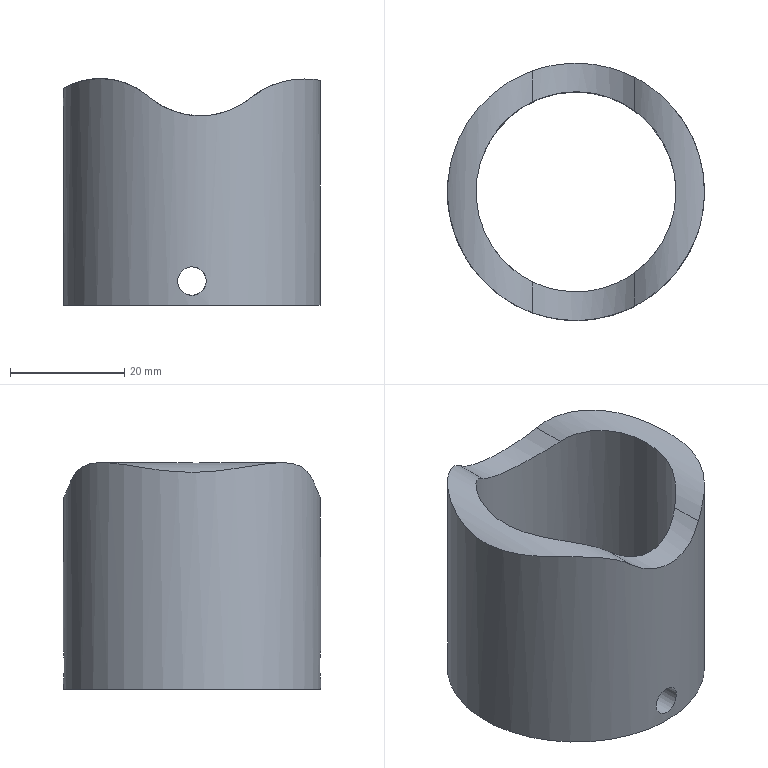Component | NX | PISTON | 1 solid | 9 faces | box 45 x 45 x 39.71 mm | volume 23430 mm3 | cylinder 8 | plane 1 | commonest cylinder face diameters 27.799 x2 5 x2 45 x1 35 x1 26.024 x1 29.489 x1
STEP:
#1=VALUE_REPRESENTATION_ITEM('',COUNT_MEASURE(0.));
#2=(LENGTH_UNIT()NAMED_UNIT(*)SI_UNIT(.MILLI.,.METRE.));
#3=UNCERTAINTY_MEASURE_WITH_UNIT(LENGTH_MEASURE(0.0508),#2,'','');
#4=(NAMED_UNIT(*)PLANE_ANGLE_UNIT()SI_UNIT($,.RADIAN.));
#5=PLANE_ANGLE_MEASURE_WITH_UNIT(PLANE_ANGLE_MEASURE(0.01745),#4);
#6=DIMENSIONAL_EXPONENTS(0.,0.,0.,0.,0.,0.,0.);
#7=(CONVERSION_BASED_UNIT('',#5)NAMED_UNIT(#6)PLANE_ANGLE_UNIT());
#8=(NAMED_UNIT(*)SI_UNIT($,.STERADIAN.)SOLID_ANGLE_UNIT());
#9=(GEOMETRIC_REPRESENTATION_CONTEXT(3)GLOBAL_UNCERTAINTY_ASSIGNED_CONTEXT((#3))GLOBAL_UNIT_ASSIGNED_CONTEXT((#2,#7,#8))REPRESENTATION_CONTEXT('',''));
#10=REPRESENTATION('',(#1),#9);
#11=VALUE_REPRESENTATION_ITEM('',COUNT_MEASURE(0.));
#12=REPRESENTATION('',(#11),#9);
#13=CARTESIAN_POINT('',(0.,0.,0.));
#14=DIRECTION('',(0.,0.,1.));
#15=DIRECTION('',(1.,0.,0.));
#16=AXIS2_PLACEMENT_3D('',#13,#14,#15);
#17=SHAPE_REPRESENTATION('',(#16),#9);
#18=CARTESIAN_POINT('',(2.606,67.362,109.935));
#19=VERTEX_POINT('',#18);
#20=CARTESIAN_POINT('',(2.606,67.362,109.935));
#21=CARTESIAN_POINT('',(2.606,67.362,110.214));
#22=CARTESIAN_POINT('',(2.558,67.368,110.497));
#23=CARTESIAN_POINT('',(2.466,67.377,110.76));
#24=CARTESIAN_POINT('',(2.374,67.387,111.023));
#25=CARTESIAN_POINT('',(2.235,67.401,111.273));
#26=CARTESIAN_POINT('',(2.062,67.416,111.491));
#27=CARTESIAN_POINT('',(1.888,67.431,111.71));
#28=CARTESIAN_POINT('',(1.674,67.447,111.902));
#29=CARTESIAN_POINT('',(1.437,67.461,112.051));
#30=CARTESIAN_POINT('',(1.2,67.475,112.2));
#31=CARTESIAN_POINT('',(0.9339,67.487,112.31));
#32=CARTESIAN_POINT('',(0.6604,67.494,112.373));
#33=CARTESIAN_POINT('',(0.388,67.5,112.435));
#34=CARTESIAN_POINT('',(0.1011,67.502,112.451));
#35=CARTESIAN_POINT('',(-0.1765,67.498,112.419));
#36=CARTESIAN_POINT('',(-0.4529,67.494,112.388));
#37=CARTESIAN_POINT('',(-0.7277,67.485,112.308));
#38=CARTESIAN_POINT('',(-0.9781,67.473,112.188));
#39=CARTESIAN_POINT('',(-1.229,67.461,112.067));
#40=CARTESIAN_POINT('',(-1.463,67.445,111.902));
#41=CARTESIAN_POINT('',(-1.66,67.43,111.705));
#42=CARTESIAN_POINT('',(-1.858,67.414,111.507));
#43=CARTESIAN_POINT('',(-2.025,67.398,111.273));
#44=CARTESIAN_POINT('',(-2.146,67.386,111.021));
#45=CARTESIAN_POINT('',(-2.268,67.373,110.768));
#46=CARTESIAN_POINT('',(-2.348,67.364,110.491));
#47=CARTESIAN_POINT('',(-2.379,67.361,110.213));
#48=CARTESIAN_POINT('',(-2.41,67.357,109.935));
#49=CARTESIAN_POINT('',(-2.394,67.359,109.649));
#50=CARTESIAN_POINT('',(-2.331,67.366,109.377));
#51=CARTESIAN_POINT('',(-2.269,67.373,109.106));
#52=CARTESIAN_POINT('',(-2.16,67.385,108.842));
#53=CARTESIAN_POINT('',(-2.012,67.399,108.607));
#54=CARTESIAN_POINT('',(-1.864,67.413,108.371));
#55=CARTESIAN_POINT('',(-1.673,67.43,108.157));
#56=CARTESIAN_POINT('',(-1.456,67.445,107.982));
#57=CARTESIAN_POINT('',(-1.237,67.46,107.807));
#58=CARTESIAN_POINT('',(-0.9845,67.474,107.668));
#59=CARTESIAN_POINT('',(-0.7198,67.484,107.575));
#60=CARTESIAN_POINT('',(-0.4557,67.494,107.483));
#61=CARTESIAN_POINT('',(-0.1718,67.5,107.435));
#62=CARTESIAN_POINT('',(0.1082,67.5,107.435));
#63=CARTESIAN_POINT('',(0.3867,67.5,107.435));
#64=CARTESIAN_POINT('',(0.6689,67.495,107.483));
#65=CARTESIAN_POINT('',(0.9316,67.485,107.575));
#66=CARTESIAN_POINT('',(1.194,67.476,107.667));
#67=CARTESIAN_POINT('',(1.444,67.462,107.806));
#68=CARTESIAN_POINT('',(1.662,67.447,107.979));
#69=CARTESIAN_POINT('',(1.881,67.432,108.153));
#70=CARTESIAN_POINT('',(2.072,67.416,108.367));
#71=CARTESIAN_POINT('',(2.221,67.402,108.603));
#72=CARTESIAN_POINT('',(2.371,67.388,108.84));
#73=CARTESIAN_POINT('',(2.481,67.376,109.107));
#74=CARTESIAN_POINT('',(2.543,67.369,109.38));
#75=CARTESIAN_POINT('',(2.585,67.365,109.562));
#76=CARTESIAN_POINT('',(2.606,67.362,109.749));
#77=CARTESIAN_POINT('',(2.606,67.362,109.935));
#78=B_SPLINE_CURVE_WITH_KNOTS('',3,(#20,#21,#22,#23,#24,#25,#26,#27,#28,#29,#30,#31,#32,#33,#34,#35,#36,#37,#38,#39,#40,#41,#42,#43,#44,#45,#46,#47,#48,#49,#50,#51,#52,#53,#54,#55,#56,#57,#58,#59,#60,#61,#62,#63,#64,#65,#66,#67,#68,#69,#70,#71,#72,#73,#74,#75,#76,#77),.UNSPECIFIED.,.T.,.F.,(1,3,3,3,3,3,3,3,3,3,3,3,3,3,3,3,3,3,3,3,3,1),(-0.0354,0.,0.05348,0.1069,0.1606,0.2144,0.268,0.3214,0.3749,0.4286,0.4824,0.5359,0.5892,0.6428,0.6966,0.7503,0.8037,0.8571,0.9108,0.9646,1.,1.053),.UNSPECIFIED.);
#79=EDGE_CURVE('',#19,#19,#78,.T.);
#80=ORIENTED_EDGE('',*,*,#79,.T.);
#81=EDGE_LOOP('',(#80));
#82=FACE_BOUND('',#81,.T.);
#83=CARTESIAN_POINT('',(0.1196,22.5,107.435));
#84=VERTEX_POINT('',#83);
#85=CARTESIAN_POINT('',(0.1196,22.5,107.435));
#86=CARTESIAN_POINT('',(-0.1592,22.5,107.434));
#87=CARTESIAN_POINT('',(-0.4422,22.505,107.48));
#88=CARTESIAN_POINT('',(-0.7058,22.515,107.57));
#89=CARTESIAN_POINT('',(-0.9693,22.525,107.661));
#90=CARTESIAN_POINT('',(-1.221,22.539,107.798));
#91=CARTESIAN_POINT('',(-1.44,22.554,107.97));
#92=CARTESIAN_POINT('',(-1.659,22.569,108.142));
#93=CARTESIAN_POINT('',(-1.852,22.586,108.355));
#94=CARTESIAN_POINT('',(-2.002,22.6,108.591));
#95=CARTESIAN_POINT('',(-2.153,22.615,108.827));
#96=CARTESIAN_POINT('',(-2.265,22.627,109.093));
#97=CARTESIAN_POINT('',(-2.329,22.634,109.366));
#98=CARTESIAN_POINT('',(-2.392,22.641,109.638));
#99=CARTESIAN_POINT('',(-2.41,22.643,109.925));
#100=CARTESIAN_POINT('',(-2.38,22.639,110.203));
#101=CARTESIAN_POINT('',(-2.35,22.636,110.48));
#102=CARTESIAN_POINT('',(-2.272,22.627,110.755));
#103=CARTESIAN_POINT('',(-2.153,22.615,111.006));
#104=CARTESIAN_POINT('',(-2.034,22.603,111.258));
#105=CARTESIAN_POINT('',(-1.87,22.587,111.492));
#106=CARTESIAN_POINT('',(-1.675,22.572,111.69));
#107=CARTESIAN_POINT('',(-1.478,22.556,111.89));
#108=CARTESIAN_POINT('',(-1.244,22.54,112.058));
#109=CARTESIAN_POINT('',(-0.9929,22.528,112.181));
#110=CARTESIAN_POINT('',(-0.7413,22.515,112.304));
#111=CARTESIAN_POINT('',(-0.4647,22.506,112.385));
#112=CARTESIAN_POINT('',(-0.1862,22.502,112.418));
#113=CARTESIAN_POINT('',(0.09079,22.498,112.451));
#114=CARTESIAN_POINT('',(0.3773,22.5,112.436));
#115=CARTESIAN_POINT('',(0.6495,22.506,112.375));
#116=CARTESIAN_POINT('',(0.9209,22.513,112.315));
#117=CARTESIAN_POINT('',(1.186,22.524,112.207));
#118=CARTESIAN_POINT('',(1.422,22.538,112.06));
#119=CARTESIAN_POINT('',(1.659,22.551,111.914));
#120=CARTESIAN_POINT('',(1.874,22.568,111.724));
#121=CARTESIAN_POINT('',(2.049,22.583,111.507));
#122=CARTESIAN_POINT('',(2.226,22.598,111.289));
#123=CARTESIAN_POINT('',(2.367,22.612,111.038));
#124=CARTESIAN_POINT('',(2.461,22.622,110.774));
#125=CARTESIAN_POINT('',(2.555,22.632,110.51));
#126=CARTESIAN_POINT('',(2.604,22.638,110.227));
#127=CARTESIAN_POINT('',(2.606,22.638,109.947));
#128=CARTESIAN_POINT('',(2.607,22.638,109.668));
#129=CARTESIAN_POINT('',(2.56,22.633,109.386));
#130=CARTESIAN_POINT('',(2.47,22.623,109.122));
#131=CARTESIAN_POINT('',(2.379,22.614,108.859));
#132=CARTESIAN_POINT('',(2.243,22.6,108.608));
#133=CARTESIAN_POINT('',(2.071,22.585,108.39));
#134=CARTESIAN_POINT('',(1.898,22.57,108.17));
#135=CARTESIAN_POINT('',(1.685,22.553,107.977));
#136=CARTESIAN_POINT('',(1.449,22.539,107.827));
#137=CARTESIAN_POINT('',(1.213,22.525,107.676));
#138=CARTESIAN_POINT('',(0.9472,22.514,107.564));
#139=CARTESIAN_POINT('',(0.674,22.507,107.501));
#140=CARTESIAN_POINT('',(0.4929,22.502,107.458));
#141=CARTESIAN_POINT('',(0.3057,22.5,107.436));
#142=CARTESIAN_POINT('',(0.1196,22.5,107.435));
#143=B_SPLINE_CURVE_WITH_KNOTS('',3,(#85,#86,#87,#88,#89,#90,#91,#92,#93,#94,#95,#96,#97,#98,#99,#100,#101,#102,#103,#104,#105,#106,#107,#108,#109,#110,#111,#112,#113,#114,#115,#116,#117,#118,#119,#120,#121,#122,#123,#124,#125,#126,#127,#128,#129,#130,#131,#132,#133,#134,#135,#136,#137,#138,#139,#140,#141,#142),.UNSPECIFIED.,.T.,.F.,(1,3,3,3,3,3,3,3,3,3,3,3,3,3,3,3,3,3,3,3,3,1),(-0.03541,0.,0.05348,0.1069,0.1606,0.2144,0.268,0.3214,0.3748,0.4286,0.4824,0.5359,0.5892,0.6428,0.6966,0.7503,0.8037,0.8571,0.9108,0.9646,1.,1.053),.UNSPECIFIED.);
#144=EDGE_CURVE('',#84,#84,#143,.T.);
#145=ORIENTED_EDGE('',*,*,#144,.T.);
#146=EDGE_LOOP('',(#145));
#147=FACE_BOUND('',#146,.T.);
#148=CARTESIAN_POINT('',(22.62,45.,105.668));
#149=VERTEX_POINT('',#148);
#150=CARTESIAN_POINT('',(0.1196,45.,105.668));
#151=DIRECTION('',(0.,0.,-1.));
#152=DIRECTION('',(1.,0.,0.));
#153=AXIS2_PLACEMENT_3D('',#150,#151,#152);
#154=CIRCLE('',#153,22.5);
#155=EDGE_CURVE('',#149,#149,#154,.T.);
#156=ORIENTED_EDGE('',*,*,#155,.F.);
#157=EDGE_LOOP('',(#156));
#158=FACE_BOUND('',#157,.T.);
#159=CARTESIAN_POINT('',(-7.471,66.181,142.211));
#160=VERTEX_POINT('',#159);
#161=CARTESIAN_POINT('',(-7.471,23.819,142.211));
#162=VERTEX_POINT('',#161);
#163=CARTESIAN_POINT('',(-7.471,66.181,142.211));
#164=CARTESIAN_POINT('',(-9.222,65.553,143.721));
#165=CARTESIAN_POINT('',(-11.257,64.552,144.637));
#166=CARTESIAN_POINT('',(-15.024,61.804,145.476));
#167=CARTESIAN_POINT('',(-16.728,60.101,145.422));
#168=CARTESIAN_POINT('',(-19.506,56.256,144.956));
#169=CARTESIAN_POINT('',(-20.553,54.188,144.559));
#170=CARTESIAN_POINT('',(-22.007,49.711,143.909));
#171=CARTESIAN_POINT('',(-22.378,47.393,143.679));
#172=CARTESIAN_POINT('',(-22.383,42.659,143.676));
#173=CARTESIAN_POINT('',(-22.012,40.312,143.906));
#174=CARTESIAN_POINT('',(-20.566,35.842,144.554));
#175=CARTESIAN_POINT('',(-19.508,33.749,144.955));
#176=CARTESIAN_POINT('',(-16.745,29.919,145.42));
#177=CARTESIAN_POINT('',(-15.033,28.204,145.477));
#178=CARTESIAN_POINT('',(-11.26,25.45,144.639));
#179=CARTESIAN_POINT('',(-9.223,24.447,143.721));
#180=CARTESIAN_POINT('',(-7.471,23.819,142.211));
#181=B_SPLINE_CURVE_WITH_KNOTS('',3,(#163,#164,#165,#166,#167,#168,#169,#170,#171,#172,#173,#174,#175,#176,#177,#178,#179,#180),.UNSPECIFIED.,.F.,.F.,(4,2,2,2,2,2,2,2,4),(0.,0.125,0.25,0.375,0.5,0.625,0.75,0.875,1.),.UNSPECIFIED.);
#182=EDGE_CURVE('',#160,#162,#181,.T.);
#183=ORIENTED_EDGE('',*,*,#182,.F.);
#184=CARTESIAN_POINT('',(10.4,65.014,141.975));
#185=VERTEX_POINT('',#184);
#186=CARTESIAN_POINT('',(10.4,65.014,141.975));
#187=CARTESIAN_POINT('',(7.997,66.248,140.011));
#188=CARTESIAN_POINT('',(4.868,67.244,138.824));
#189=CARTESIAN_POINT('',(-1.777,67.666,138.853));
#190=CARTESIAN_POINT('',(-5.027,67.057,140.103));
#191=CARTESIAN_POINT('',(-7.471,66.181,142.211));
#192=B_SPLINE_CURVE_WITH_KNOTS('',3,(#186,#187,#188,#189,#190,#191),.UNSPECIFIED.,.F.,.F.,(4,2,4),(0.,0.5,1.),.UNSPECIFIED.);
#193=EDGE_CURVE('',#185,#160,#192,.T.);
#194=ORIENTED_EDGE('',*,*,#193,.F.);
#195=CARTESIAN_POINT('',(10.4,24.986,141.975));
#196=VERTEX_POINT('',#195);
#197=CARTESIAN_POINT('',(10.4,24.986,141.975));
#198=CARTESIAN_POINT('',(11.936,25.775,143.23));
#199=CARTESIAN_POINT('',(13.594,26.864,144.06));
#200=CARTESIAN_POINT('',(16.65,29.599,145.066));
#201=CARTESIAN_POINT('',(18.043,31.238,145.247));
#202=CARTESIAN_POINT('',(21.397,36.566,145.377));
#203=CARTESIAN_POINT('',(22.621,40.804,145.015));
#204=CARTESIAN_POINT('',(22.619,47.109,145.016));
#205=CARTESIAN_POINT('',(22.324,49.204,145.083));
#206=CARTESIAN_POINT('',(21.153,53.266,145.245));
#207=CARTESIAN_POINT('',(20.298,55.178,145.334));
#208=CARTESIAN_POINT('',(18.043,58.765,145.248));
#209=CARTESIAN_POINT('',(16.675,60.377,145.073));
#210=CARTESIAN_POINT('',(13.591,63.14,144.061));
#211=CARTESIAN_POINT('',(11.937,64.225,143.23));
#212=CARTESIAN_POINT('',(10.4,65.014,141.975));
#213=B_SPLINE_CURVE_WITH_KNOTS('',3,(#197,#198,#199,#200,#201,#202,#203,#204,#205,#206,#207,#208,#209,#210,#211,#212),.UNSPECIFIED.,.F.,.F.,(4,2,2,2,2,2,2,4),(0.,0.125,0.25,0.5,0.625,0.75,0.875,1.),.UNSPECIFIED.);
#214=EDGE_CURVE('',#196,#185,#213,.T.);
#215=ORIENTED_EDGE('',*,*,#214,.F.);
#216=CARTESIAN_POINT('',(-7.471,23.819,142.211));
#217=CARTESIAN_POINT('',(-6.251,23.382,141.158));
#218=CARTESIAN_POINT('',(-4.857,23.002,140.323));
#219=CARTESIAN_POINT('',(-1.782,22.527,139.157));
#220=CARTESIAN_POINT('',(-0.1319,22.441,138.849));
#221=CARTESIAN_POINT('',(4.825,22.75,138.818));
#222=CARTESIAN_POINT('',(7.996,23.751,140.01));
#223=CARTESIAN_POINT('',(10.4,24.986,141.975));
#224=B_SPLINE_CURVE_WITH_KNOTS('',3,(#216,#217,#218,#219,#220,#221,#222,#223),.UNSPECIFIED.,.F.,.F.,(4,2,2,4),(0.,0.25,0.5,1.),.UNSPECIFIED.);
#225=EDGE_CURVE('',#162,#196,#224,.T.);
#226=ORIENTED_EDGE('',*,*,#225,.F.);
#227=EDGE_LOOP('',(#183,#194,#215,#226));
#228=FACE_BOUND('',#227,.T.);
#229=CARTESIAN_POINT('',(0.1196,45.,105.668));
#230=DIRECTION('',(0.,0.,1.));
#231=DIRECTION('',(0.,-1.,0.));
#232=AXIS2_PLACEMENT_3D('',#229,#230,#231);
#233=CYLINDRICAL_SURFACE('',#232,22.5);
#234=ADVANCED_FACE('',(#82,#147,#158,#228),#233,.T.);
#235=CARTESIAN_POINT('',(0.1196,27.5,107.435));
#236=VERTEX_POINT('',#235);
#237=CARTESIAN_POINT('',(0.1196,27.5,107.435));
#238=CARTESIAN_POINT('',(-0.1586,27.5,107.434));
#239=CARTESIAN_POINT('',(-0.4409,27.507,107.48));
#240=CARTESIAN_POINT('',(-0.7039,27.519,107.57));
#241=CARTESIAN_POINT('',(-0.9668,27.532,107.66));
#242=CARTESIAN_POINT('',(-1.218,27.55,107.796));
#243=CARTESIAN_POINT('',(-1.436,27.569,107.967));
#244=CARTESIAN_POINT('',(-1.656,27.589,108.139));
#245=CARTESIAN_POINT('',(-1.849,27.61,108.351));
#246=CARTESIAN_POINT('',(-2.,27.629,108.587));
#247=CARTESIAN_POINT('',(-2.151,27.647,108.823));
#248=CARTESIAN_POINT('',(-2.264,27.663,109.089));
#249=CARTESIAN_POINT('',(-2.328,27.672,109.362));
#250=CARTESIAN_POINT('',(-2.392,27.681,109.634));
#251=CARTESIAN_POINT('',(-2.41,27.684,109.921));
#252=CARTESIAN_POINT('',(-2.381,27.68,110.198));
#253=CARTESIAN_POINT('',(-2.351,27.675,110.474));
#254=CARTESIAN_POINT('',(-2.275,27.664,110.748));
#255=CARTESIAN_POINT('',(-2.157,27.649,110.999));
#256=CARTESIAN_POINT('',(-2.039,27.633,111.25));
#257=CARTESIAN_POINT('',(-1.876,27.613,111.484));
#258=CARTESIAN_POINT('',(-1.682,27.593,111.682));
#259=CARTESIAN_POINT('',(-1.487,27.573,111.883));
#260=CARTESIAN_POINT('',(-1.254,27.552,112.052));
#261=CARTESIAN_POINT('',(-1.003,27.536,112.176));
#262=CARTESIAN_POINT('',(-0.7514,27.52,112.3));
#263=CARTESIAN_POINT('',(-0.4748,27.508,112.383));
#264=CARTESIAN_POINT('',(-0.1961,27.503,112.417));
#265=CARTESIAN_POINT('',(0.08026,27.498,112.45));
#266=CARTESIAN_POINT('',(0.3663,27.5,112.437));
#267=CARTESIAN_POINT('',(0.6382,27.508,112.378));
#268=CARTESIAN_POINT('',(0.9089,27.516,112.319));
#269=CARTESIAN_POINT('',(1.173,27.53,112.213));
#270=CARTESIAN_POINT('',(1.409,27.548,112.068));
#271=CARTESIAN_POINT('',(1.646,27.565,111.923));
#272=CARTESIAN_POINT('',(1.862,27.586,111.736));
#273=CARTESIAN_POINT('',(2.039,27.606,111.52));
#274=CARTESIAN_POINT('',(2.216,27.625,111.304));
#275=CARTESIAN_POINT('',(2.359,27.644,111.053));
#276=CARTESIAN_POINT('',(2.455,27.657,110.789));
#277=CARTESIAN_POINT('',(2.551,27.669,110.526));
#278=CARTESIAN_POINT('',(2.602,27.677,110.243));
#279=CARTESIAN_POINT('',(2.605,27.677,109.962));
#280=CARTESIAN_POINT('',(2.608,27.678,109.685));
#281=CARTESIAN_POINT('',(2.564,27.671,109.403));
#282=CARTESIAN_POINT('',(2.476,27.659,109.14));
#283=CARTESIAN_POINT('',(2.388,27.647,108.877));
#284=CARTESIAN_POINT('',(2.253,27.63,108.626));
#285=CARTESIAN_POINT('',(2.084,27.611,108.407));
#286=CARTESIAN_POINT('',(1.914,27.591,108.186));
#287=CARTESIAN_POINT('',(1.703,27.57,107.991));
#288=CARTESIAN_POINT('',(1.468,27.552,107.839));
#289=CARTESIAN_POINT('',(1.233,27.534,107.686));
#290=CARTESIAN_POINT('',(0.9681,27.518,107.572));
#291=CARTESIAN_POINT('',(0.6951,27.509,107.506));
#292=CARTESIAN_POINT('',(0.5074,27.503,107.46));
#293=CARTESIAN_POINT('',(0.3129,27.5,107.436));
#294=CARTESIAN_POINT('',(0.1196,27.5,107.435));
#295=B_SPLINE_CURVE_WITH_KNOTS('',3,(#237,#238,#239,#240,#241,#242,#243,#244,#245,#246,#247,#248,#249,#250,#251,#252,#253,#254,#255,#256,#257,#258,#259,#260,#261,#262,#263,#264,#265,#266,#267,#268,#269,#270,#271,#272,#273,#274,#275,#276,#277,#278,#279,#280,#281,#282,#283,#284,#285,#286,#287,#288,#289,#290,#291,#292,#293,#294),.UNSPECIFIED.,.T.,.F.,(1,3,3,3,3,3,3,3,3,3,3,3,3,3,3,3,3,3,3,3,3,1),(-0.03677,0.,0.05333,0.1066,0.1603,0.2142,0.2677,0.3208,0.3741,0.4279,0.4818,0.5351,0.5883,0.6417,0.6956,0.7493,0.8025,0.8557,0.9093,0.9632,1.,1.053),.UNSPECIFIED.);
#296=EDGE_CURVE('',#236,#236,#295,.T.);
#297=ORIENTED_EDGE('',*,*,#296,.F.);
#298=EDGE_LOOP('',(#297));
#299=FACE_BOUND('',#298,.T.);
#300=CARTESIAN_POINT('',(2.606,62.323,109.935));
#301=VERTEX_POINT('',#300);
#302=CARTESIAN_POINT('',(2.606,62.323,109.935));
#303=CARTESIAN_POINT('',(2.606,62.323,110.213));
#304=CARTESIAN_POINT('',(2.558,62.33,110.495));
#305=CARTESIAN_POINT('',(2.466,62.342,110.758));
#306=CARTESIAN_POINT('',(2.375,62.354,111.02));
#307=CARTESIAN_POINT('',(2.237,62.372,111.27));
#308=CARTESIAN_POINT('',(2.065,62.392,111.488));
#309=CARTESIAN_POINT('',(1.891,62.411,111.707));
#310=CARTESIAN_POINT('',(1.678,62.432,111.899));
#311=CARTESIAN_POINT('',(1.442,62.45,112.048));
#312=CARTESIAN_POINT('',(1.205,62.468,112.198));
#313=CARTESIAN_POINT('',(0.9382,62.483,112.309));
#314=CARTESIAN_POINT('',(0.6644,62.492,112.372));
#315=CARTESIAN_POINT('',(0.3924,62.5,112.434));
#316=CARTESIAN_POINT('',(0.1057,62.502,112.451));
#317=CARTESIAN_POINT('',(-0.1718,62.498,112.42));
#318=CARTESIAN_POINT('',(-0.4472,62.493,112.389));
#319=CARTESIAN_POINT('',(-0.721,62.482,112.311));
#320=CARTESIAN_POINT('',(-0.9708,62.466,112.191));
#321=CARTESIAN_POINT('',(-1.221,62.45,112.072));
#322=CARTESIAN_POINT('',(-1.455,62.43,111.908));
#323=CARTESIAN_POINT('',(-1.652,62.41,111.713));
#324=CARTESIAN_POINT('',(-1.851,62.39,111.516));
#325=CARTESIAN_POINT('',(-2.019,62.369,111.282));
#326=CARTESIAN_POINT('',(-2.142,62.353,111.03));
#327=CARTESIAN_POINT('',(-2.265,62.337,110.778));
#328=CARTESIAN_POINT('',(-2.346,62.326,110.501));
#329=CARTESIAN_POINT('',(-2.378,62.321,110.222));
#330=CARTESIAN_POINT('',(-2.41,62.316,109.946));
#331=CARTESIAN_POINT('',(-2.395,62.319,109.66));
#332=CARTESIAN_POINT('',(-2.334,62.327,109.388));
#333=CARTESIAN_POINT('',(-2.273,62.336,109.118));
#334=CARTESIAN_POINT('',(-2.166,62.351,108.855));
#335=CARTESIAN_POINT('',(-2.02,62.369,108.62));
#336=CARTESIAN_POINT('',(-1.874,62.387,108.383));
#337=CARTESIAN_POINT('',(-1.685,62.408,108.168));
#338=CARTESIAN_POINT('',(-1.469,62.428,107.993));
#339=CARTESIAN_POINT('',(-1.251,62.448,107.816));
#340=CARTESIAN_POINT('',(-0.9995,62.466,107.675));
#341=CARTESIAN_POINT('',(-0.7351,62.479,107.581));
#342=CARTESIAN_POINT('',(-0.4715,62.492,107.487));
#343=CARTESIAN_POINT('',(-0.1877,62.5,107.437));
#344=CARTESIAN_POINT('',(0.09239,62.5,107.435));
#345=CARTESIAN_POINT('',(0.37,62.5,107.434));
#346=CARTESIAN_POINT('',(0.6517,62.494,107.48));
#347=CARTESIAN_POINT('',(0.9142,62.482,107.569));
#348=CARTESIAN_POINT('',(1.177,62.47,107.659));
#349=CARTESIAN_POINT('',(1.427,62.452,107.795));
#350=CARTESIAN_POINT('',(1.645,62.433,107.965));
#351=CARTESIAN_POINT('',(1.865,62.414,108.137));
#352=CARTESIAN_POINT('',(2.058,62.393,108.349));
#353=CARTESIAN_POINT('',(2.209,62.375,108.584));
#354=CARTESIAN_POINT('',(2.361,62.357,108.82));
#355=CARTESIAN_POINT('',(2.474,62.341,109.086));
#356=CARTESIAN_POINT('',(2.538,62.332,109.359));
#357=CARTESIAN_POINT('',(2.583,62.326,109.547));
#358=CARTESIAN_POINT('',(2.606,62.323,109.742));
#359=CARTESIAN_POINT('',(2.606,62.323,109.935));
#360=B_SPLINE_CURVE_WITH_KNOTS('',3,(#302,#303,#304,#305,#306,#307,#308,#309,#310,#311,#312,#313,#314,#315,#316,#317,#318,#319,#320,#321,#322,#323,#324,#325,#326,#327,#328,#329,#330,#331,#332,#333,#334,#335,#336,#337,#338,#339,#340,#341,#342,#343,#344,#345,#346,#347,#348,#349,#350,#351,#352,#353,#354,#355,#356,#357,#358,#359),.UNSPECIFIED.,.T.,.F.,(1,3,3,3,3,3,3,3,3,3,3,3,3,3,3,3,3,3,3,3,3,1),(-0.03676,0.,0.05333,0.1066,0.1603,0.2142,0.2677,0.3208,0.3742,0.428,0.4818,0.5351,0.5882,0.6417,0.6956,0.7493,0.8025,0.8557,0.9093,0.9632,1.,1.053),.UNSPECIFIED.);
#361=EDGE_CURVE('',#301,#301,#360,.T.);
#362=ORIENTED_EDGE('',*,*,#361,.F.);
#363=EDGE_LOOP('',(#362));
#364=FACE_BOUND('',#363,.T.);
#365=CARTESIAN_POINT('',(17.62,45.,105.668));
#366=VERTEX_POINT('',#365);
#367=CARTESIAN_POINT('',(0.1196,45.,105.668));
#368=DIRECTION('',(0.,0.,-1.));
#369=DIRECTION('',(1.,0.,0.));
#370=AXIS2_PLACEMENT_3D('',#367,#368,#369);
#371=CIRCLE('',#370,17.5);
#372=EDGE_CURVE('',#366,#366,#371,.T.);
#373=ORIENTED_EDGE('',*,*,#372,.T.);
#374=EDGE_LOOP('',(#373));
#375=FACE_BOUND('',#374,.T.);
#376=CARTESIAN_POINT('',(10.4,59.162,141.975));
#377=VERTEX_POINT('',#376);
#378=CARTESIAN_POINT('',(-7.471,60.768,142.211));
#379=VERTEX_POINT('',#378);
#380=CARTESIAN_POINT('',(10.4,59.162,141.975));
#381=CARTESIAN_POINT('',(9.253,59.995,141.037));
#382=CARTESIAN_POINT('',(7.942,60.736,140.265));
#383=CARTESIAN_POINT('',(4.954,61.895,139.154));
#384=CARTESIAN_POINT('',(3.301,62.29,138.841));
#385=CARTESIAN_POINT('',(-0.04548,62.58,138.836));
#386=CARTESIAN_POINT('',(-1.75,62.471,139.148));
#387=CARTESIAN_POINT('',(-4.852,61.853,140.318));
#388=CARTESIAN_POINT('',(-6.26,61.351,141.167));
#389=CARTESIAN_POINT('',(-7.471,60.768,142.211));
#390=B_SPLINE_CURVE_WITH_KNOTS('',3,(#380,#381,#382,#383,#384,#385,#386,#387,#388,#389),.UNSPECIFIED.,.F.,.F.,(4,2,2,2,4),(0.,0.25,0.5,0.75,1.),.UNSPECIFIED.);
#391=EDGE_CURVE('',#377,#379,#390,.T.);
#392=ORIENTED_EDGE('',*,*,#391,.T.);
#393=CARTESIAN_POINT('',(-7.471,29.232,142.211));
#394=VERTEX_POINT('',#393);
#395=CARTESIAN_POINT('',(-7.471,60.768,142.211));
#396=CARTESIAN_POINT('',(-8.687,60.183,143.259));
#397=CARTESIAN_POINT('',(-10.004,59.366,143.996));
#398=CARTESIAN_POINT('',(-12.47,57.263,144.958));
#399=CARTESIAN_POINT('',(-13.607,55.985,145.185));
#400=CARTESIAN_POINT('',(-16.371,51.756,145.493));
#401=CARTESIAN_POINT('',(-17.381,48.354,145.291));
#402=CARTESIAN_POINT('',(-17.38,41.64,145.291));
#403=CARTESIAN_POINT('',(-16.379,38.258,145.493));
#404=CARTESIAN_POINT('',(-13.611,34.019,145.186));
#405=CARTESIAN_POINT('',(-12.478,32.746,144.961));
#406=CARTESIAN_POINT('',(-10.016,30.642,144.002));
#407=CARTESIAN_POINT('',(-8.687,29.817,143.259));
#408=CARTESIAN_POINT('',(-7.471,29.232,142.211));
#409=B_SPLINE_CURVE_WITH_KNOTS('',3,(#395,#396,#397,#398,#399,#400,#401,#402,#403,#404,#405,#406,#407,#408),.UNSPECIFIED.,.F.,.F.,(4,2,2,2,2,2,4),(0.,0.125,0.25,0.5,0.75,0.875,1.),.UNSPECIFIED.);
#410=EDGE_CURVE('',#379,#394,#409,.T.);
#411=ORIENTED_EDGE('',*,*,#410,.T.);
#412=CARTESIAN_POINT('',(10.4,30.838,141.975));
#413=VERTEX_POINT('',#412);
#414=CARTESIAN_POINT('',(-7.471,29.232,142.211));
#415=CARTESIAN_POINT('',(-6.261,28.649,141.167));
#416=CARTESIAN_POINT('',(-4.862,28.15,140.323));
#417=CARTESIAN_POINT('',(-1.759,27.529,139.15));
#418=CARTESIAN_POINT('',(-0.06403,27.42,138.838));
#419=CARTESIAN_POINT('',(3.287,27.707,138.839));
#420=CARTESIAN_POINT('',(4.946,28.103,139.153));
#421=CARTESIAN_POINT('',(7.922,29.255,140.255));
#422=CARTESIAN_POINT('',(9.252,30.005,141.036));
#423=CARTESIAN_POINT('',(10.4,30.838,141.975));
#424=B_SPLINE_CURVE_WITH_KNOTS('',3,(#414,#415,#416,#417,#418,#419,#420,#421,#422,#423),.UNSPECIFIED.,.F.,.F.,(4,2,2,2,4),(0.,0.25,0.5,0.75,1.),.UNSPECIFIED.);
#425=EDGE_CURVE('',#394,#413,#424,.T.);
#426=ORIENTED_EDGE('',*,*,#425,.T.);
#427=CARTESIAN_POINT('',(10.4,30.838,141.975));
#428=CARTESIAN_POINT('',(12.339,32.246,143.559));
#429=CARTESIAN_POINT('',(14.274,34.329,144.324));
#430=CARTESIAN_POINT('',(16.914,39.326,145.095));
#431=CARTESIAN_POINT('',(17.621,42.181,145.15));
#432=CARTESIAN_POINT('',(17.618,47.833,145.15));
#433=CARTESIAN_POINT('',(16.921,50.659,145.097));
#434=CARTESIAN_POINT('',(14.932,54.426,144.516));
#435=CARTESIAN_POINT('',(14.14,55.558,144.237));
#436=CARTESIAN_POINT('',(12.362,57.577,143.367));
#437=CARTESIAN_POINT('',(11.37,58.458,142.767));
#438=CARTESIAN_POINT('',(10.4,59.162,141.975));
#439=B_SPLINE_CURVE_WITH_KNOTS('',3,(#427,#428,#429,#430,#431,#432,#433,#434,#435,#436,#437,#438),.UNSPECIFIED.,.F.,.F.,(4,2,2,2,2,4),(0.,0.25,0.5,0.75,0.875,1.),.UNSPECIFIED.);
#440=EDGE_CURVE('',#413,#377,#439,.T.);
#441=ORIENTED_EDGE('',*,*,#440,.T.);
#442=EDGE_LOOP('',(#392,#411,#426,#441));
#443=FACE_BOUND('',#442,.T.);
#444=CARTESIAN_POINT('',(0.1196,45.,105.668));
#445=DIRECTION('',(0.,0.,1.));
#446=DIRECTION('',(0.,-1.,0.));
#447=AXIS2_PLACEMENT_3D('',#444,#445,#446);
#448=CYLINDRICAL_SURFACE('',#447,17.5);
#449=ADVANCED_FACE('',(#299,#364,#375,#443),#448,.F.);
#450=ORIENTED_EDGE('',*,*,#155,.T.);
#451=EDGE_LOOP('',(#450));
#452=FACE_BOUND('',#451,.T.);
#453=ORIENTED_EDGE('',*,*,#372,.F.);
#454=EDGE_LOOP('',(#453));
#455=FACE_BOUND('',#454,.T.);
#456=CARTESIAN_POINT('',(0.1196,45.,105.668));
#457=DIRECTION('',(0.,0.,-1.));
#458=DIRECTION('',(0.,1.,0.));
#459=AXIS2_PLACEMENT_3D('',#456,#457,#458);
#460=PLANE('',#459);
#461=ADVANCED_FACE('',(#452,#455),#460,.T.);
#462=ORIENTED_EDGE('',*,*,#182,.T.);
#463=CARTESIAN_POINT('',(-7.471,0.,142.211));
#464=DIRECTION('',(0.,-1.,0.));
#465=VECTOR('',#464,1.);
#466=LINE('',#463,#465);
#467=EDGE_CURVE('',#394,#162,#466,.T.);
#468=ORIENTED_EDGE('',*,*,#467,.F.);
#469=ORIENTED_EDGE('',*,*,#410,.F.);
#470=CARTESIAN_POINT('',(-7.471,0.,142.211));
#471=DIRECTION('',(0.,-1.,0.));
#472=VECTOR('',#471,1.);
#473=LINE('',#470,#472);
#474=EDGE_CURVE('',#160,#379,#473,.T.);
#475=ORIENTED_EDGE('',*,*,#474,.F.);
#476=EDGE_LOOP('',(#462,#468,#469,#475));
#477=FACE_OUTER_BOUND('',#476,.T.);
#478=CARTESIAN_POINT('',(-15.968,0.,132.356));
#479=DIRECTION('',(0.,1.,0.));
#480=DIRECTION('',(-1.,0.,0.));
#481=AXIS2_PLACEMENT_3D('',#478,#479,#480);
#482=CYLINDRICAL_SURFACE('',#481,13.012);
#483=ADVANCED_FACE('',(#477),#482,.T.);
#484=ORIENTED_EDGE('',*,*,#225,.T.);
#485=CARTESIAN_POINT('',(10.4,0.,141.975));
#486=DIRECTION('',(0.,-1.,0.));
#487=VECTOR('',#486,1.);
#488=LINE('',#485,#487);
#489=EDGE_CURVE('',#413,#196,#488,.T.);
#490=ORIENTED_EDGE('',*,*,#489,.F.);
#491=ORIENTED_EDGE('',*,*,#425,.F.);
#492=ORIENTED_EDGE('',*,*,#467,.T.);
#493=EDGE_LOOP('',(#484,#490,#491,#492));
#494=FACE_OUTER_BOUND('',#493,.T.);
#495=CARTESIAN_POINT('',(1.605,0.,152.738));
#496=DIRECTION('',(0.,1.,0.));
#497=DIRECTION('',(-1.,0.,0.));
#498=AXIS2_PLACEMENT_3D('',#495,#496,#497);
#499=CYLINDRICAL_SURFACE('',#498,13.9);
#500=ADVANCED_FACE('',(#494),#499,.F.);
#501=ORIENTED_EDGE('',*,*,#193,.T.);
#502=ORIENTED_EDGE('',*,*,#474,.T.);
#503=ORIENTED_EDGE('',*,*,#391,.F.);
#504=CARTESIAN_POINT('',(10.4,0.,141.975));
#505=DIRECTION('',(0.,-1.,0.));
#506=VECTOR('',#505,1.);
#507=LINE('',#504,#506);
#508=EDGE_CURVE('',#185,#377,#507,.T.);
#509=ORIENTED_EDGE('',*,*,#508,.F.);
#510=EDGE_LOOP('',(#501,#502,#503,#509));
#511=FACE_OUTER_BOUND('',#510,.T.);
#512=CARTESIAN_POINT('',(1.605,0.,152.738));
#513=DIRECTION('',(0.,1.,0.));
#514=DIRECTION('',(-1.,0.,0.));
#515=AXIS2_PLACEMENT_3D('',#512,#513,#514);
#516=CYLINDRICAL_SURFACE('',#515,13.9);
#517=ADVANCED_FACE('',(#511),#516,.F.);
#518=ORIENTED_EDGE('',*,*,#214,.T.);
#519=ORIENTED_EDGE('',*,*,#508,.T.);
#520=ORIENTED_EDGE('',*,*,#440,.F.);
#521=ORIENTED_EDGE('',*,*,#489,.T.);
#522=EDGE_LOOP('',(#518,#519,#520,#521));
#523=FACE_OUTER_BOUND('',#522,.T.);
#524=CARTESIAN_POINT('',(19.73,0.,130.557));
#525=DIRECTION('',(0.,1.,0.));
#526=DIRECTION('',(-1.,0.,0.));
#527=AXIS2_PLACEMENT_3D('',#524,#525,#526);
#528=CYLINDRICAL_SURFACE('',#527,14.745);
#529=ADVANCED_FACE('',(#523),#528,.T.);
#530=ORIENTED_EDGE('',*,*,#361,.T.);
#531=EDGE_LOOP('',(#530));
#532=FACE_BOUND('',#531,.T.);
#533=ORIENTED_EDGE('',*,*,#79,.F.);
#534=EDGE_LOOP('',(#533));
#535=FACE_BOUND('',#534,.T.);
#536=CARTESIAN_POINT('',(0.1056,75.5,109.935));
#537=DIRECTION('',(0.,-1.,0.));
#538=DIRECTION('',(1.,0.,0.));
#539=AXIS2_PLACEMENT_3D('',#536,#537,#538);
#540=CYLINDRICAL_SURFACE('',#539,2.5);
#541=ADVANCED_FACE('',(#532,#535),#540,.F.);
#542=ORIENTED_EDGE('',*,*,#296,.T.);
#543=EDGE_LOOP('',(#542));
#544=FACE_BOUND('',#543,.T.);
#545=ORIENTED_EDGE('',*,*,#144,.F.);
#546=EDGE_LOOP('',(#545));
#547=FACE_BOUND('',#546,.T.);
#548=CARTESIAN_POINT('',(0.1056,75.5,109.935));
#549=DIRECTION('',(0.,-1.,0.));
#550=DIRECTION('',(1.,0.,0.));
#551=AXIS2_PLACEMENT_3D('',#548,#549,#550);
#552=CYLINDRICAL_SURFACE('',#551,2.5);
#553=ADVANCED_FACE('',(#544,#547),#552,.F.);
#554=CLOSED_SHELL('',(#234,#449,#461,#483,#500,#517,#529,#541,#553));
#555=MANIFOLD_SOLID_BREP('',#554);
#556=ADVANCED_BREP_SHAPE_REPRESENTATION('',(#555),#9);
#557=SHAPE_REPRESENTATION_RELATIONSHIP('','',#17,#556);
#558=PRESENTATION_LAYER_ASSIGNMENT('','',(#555));
#559=COLOUR_RGB('',0.3176,0.1216,0.498);
#560=FILL_AREA_STYLE_COLOUR('',#559);
#561=FILL_AREA_STYLE('',(#560));
#562=SURFACE_STYLE_FILL_AREA(#561);
#563=SURFACE_SIDE_STYLE('',(#562));
#564=SURFACE_STYLE_USAGE(.BOTH.,#563);
#565=PRESENTATION_STYLE_ASSIGNMENT((#564));
#566=STYLED_ITEM('',(#565),#555);
#567=MECHANICAL_DESIGN_GEOMETRIC_PRESENTATION_REPRESENTATION('',(#566),#9);